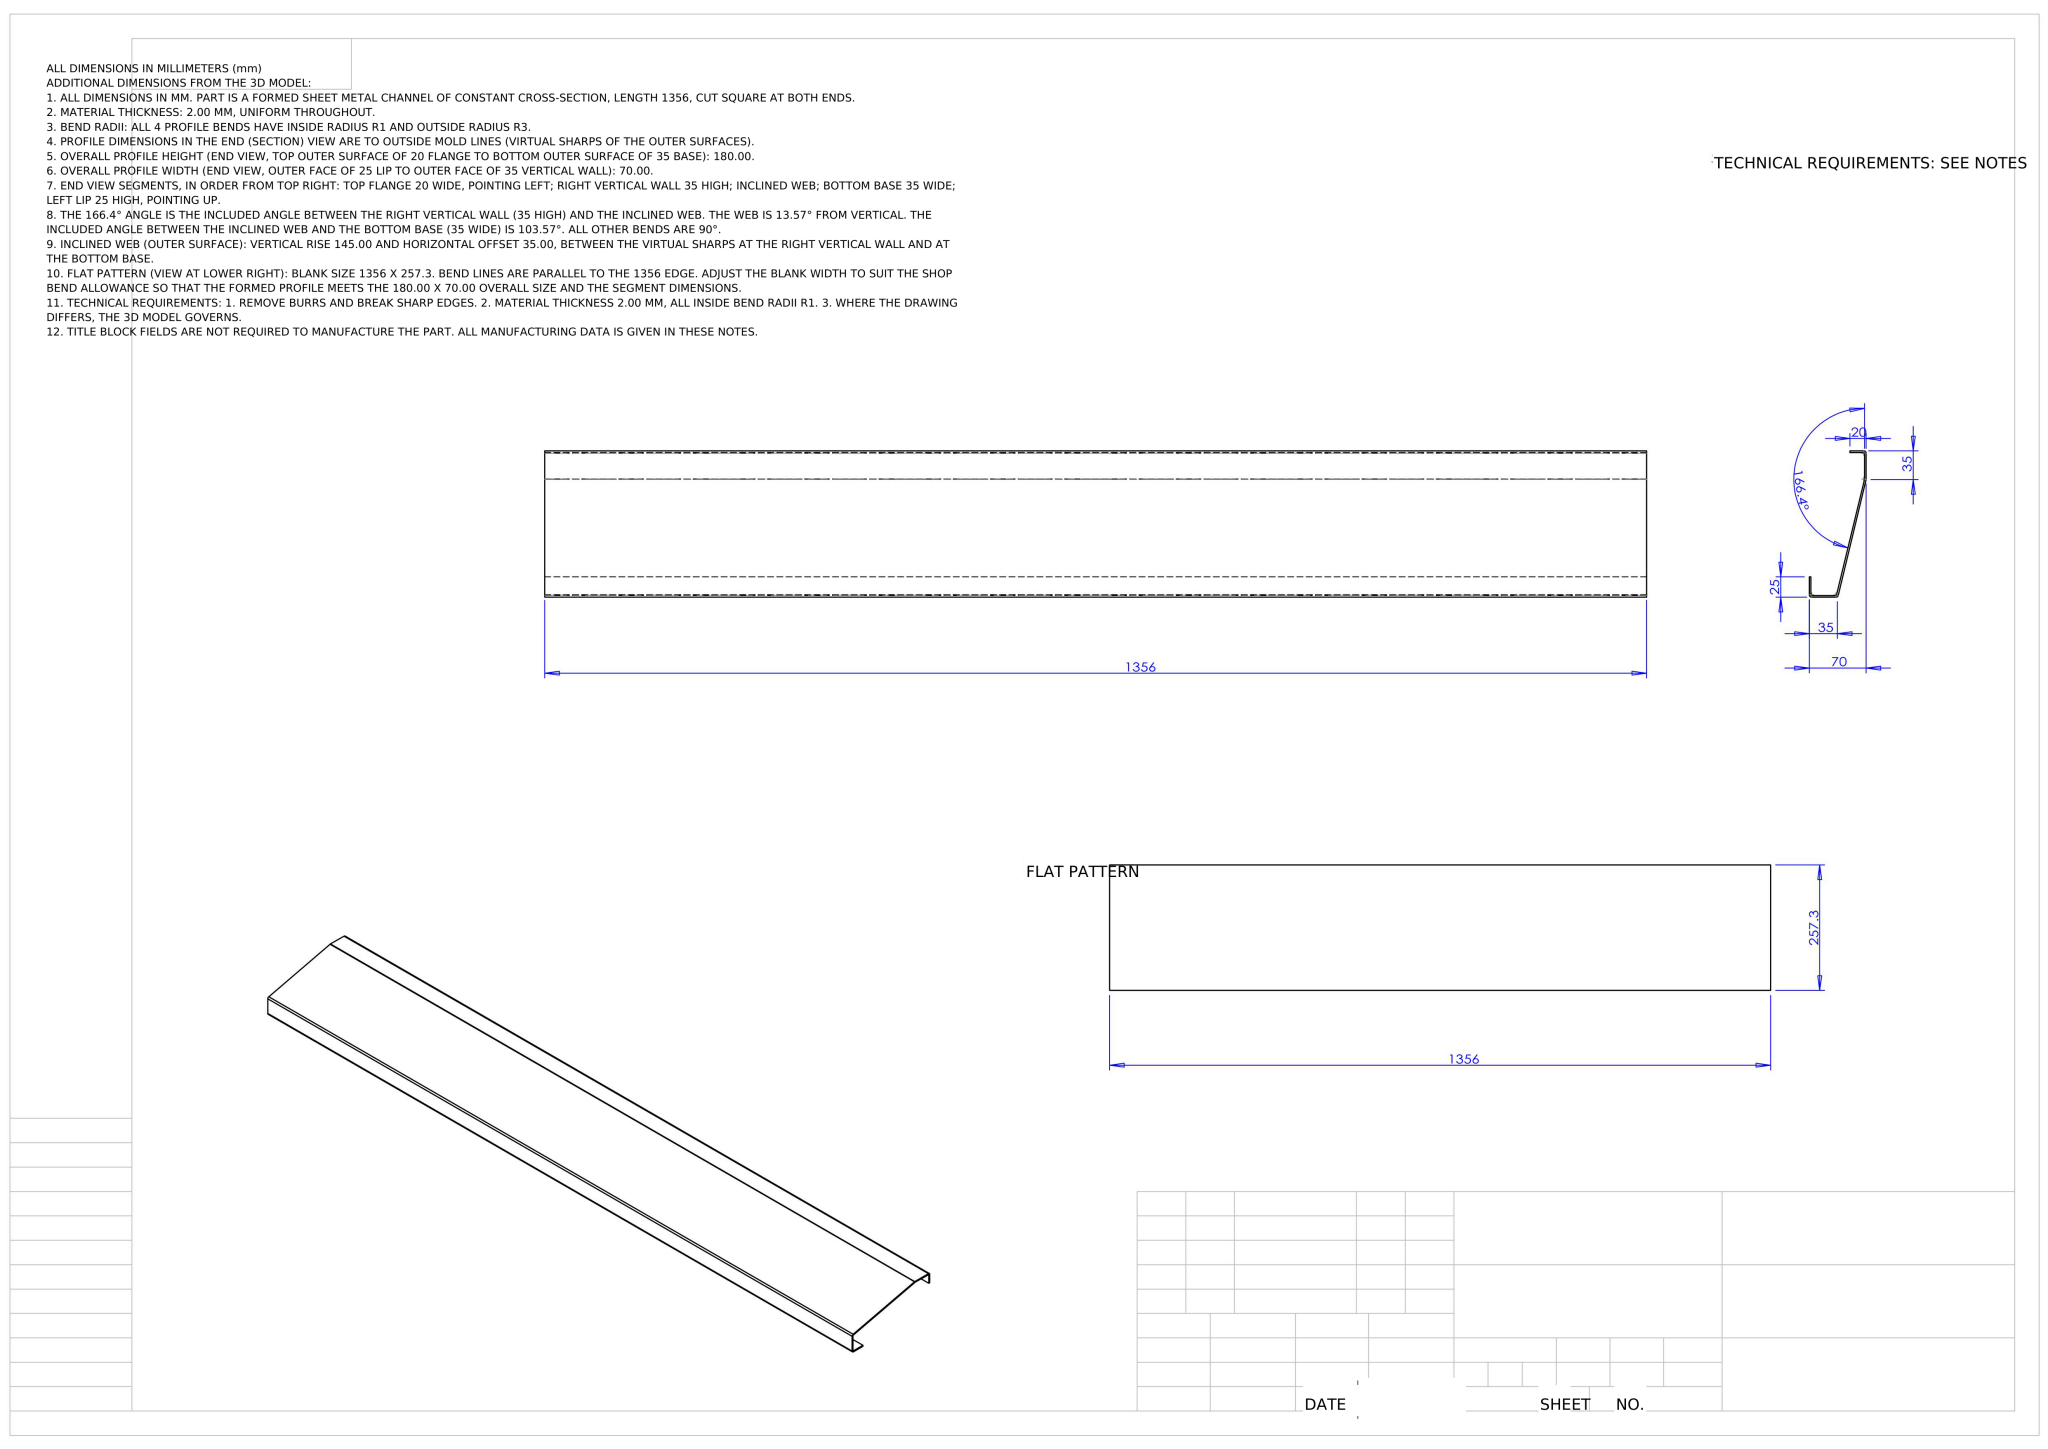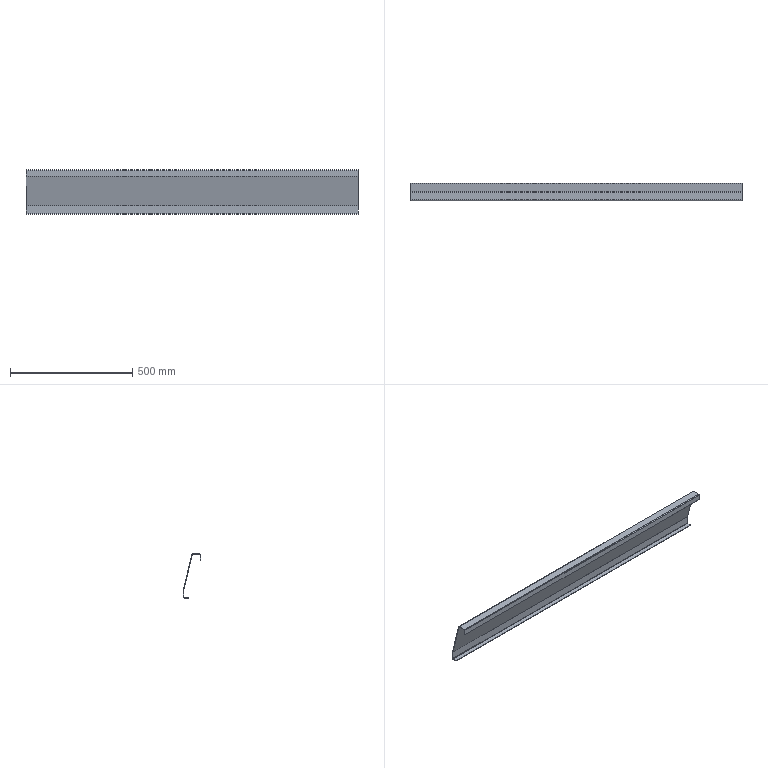Part | NX | mm | 1 solid | 38 faces | box 1356 x 70 x 180 mm | volume 694682 mm3 | plane 30 | cylinder 8 | commonest cylinder face diameters 2 x4 6 x4
STEP:
#1=COLOUR_RGB('',0.7529,0.7529,0.7529);
#2=FILL_AREA_STYLE_COLOUR('',#1);
#3=FILL_AREA_STYLE('',(#2));
#4=SURFACE_STYLE_FILL_AREA(#3);
#5=SURFACE_SIDE_STYLE('',(#4));
#6=SURFACE_STYLE_USAGE(.BOTH.,#5);
#7=PRESENTATION_STYLE_ASSIGNMENT((#6));
#8=CARTESIAN_POINT('',(1356.,-0.06513,-82.562));
#9=VERTEX_POINT('',#8);
#10=CARTESIAN_POINT('',(1356.,-0.06513,-80.562));
#11=VERTEX_POINT('',#10);
#12=CARTESIAN_POINT('',(1356.,-0.06513,-82.562));
#13=DIRECTION('',(0.,-0.,1.));
#14=VECTOR('',#13,1000.);
#15=LINE('',#12,#14);
#16=EDGE_CURVE('',#9,#11,#15,.T.);
#17=ORIENTED_EDGE('',*,*,#16,.F.);
#18=CARTESIAN_POINT('',(1356.,2.935,-79.562));
#19=VERTEX_POINT('',#18);
#20=CARTESIAN_POINT('',(1356.,-0.06513,-79.562));
#21=DIRECTION('',(1.,0.,0.));
#22=DIRECTION('',(0.,0.,1.));
#23=AXIS2_PLACEMENT_3D('',#20,#21,#22);
#24=CIRCLE('',#23,3.);
#25=EDGE_CURVE('',#9,#19,#24,.T.);
#26=ORIENTED_EDGE('',*,*,#25,.T.);
#27=CARTESIAN_POINT('',(1356.,0.9349,-79.562));
#28=VERTEX_POINT('',#27);
#29=CARTESIAN_POINT('',(1356.,0.9349,-79.562));
#30=DIRECTION('',(0.,1.,0.));
#31=VECTOR('',#30,1000.);
#32=LINE('',#29,#31);
#33=EDGE_CURVE('',#28,#19,#32,.T.);
#34=ORIENTED_EDGE('',*,*,#33,.F.);
#35=CARTESIAN_POINT('',(1356.,-0.06513,-79.562));
#36=DIRECTION('',(1.,0.,0.));
#37=DIRECTION('',(0.,0.,-1.));
#38=AXIS2_PLACEMENT_3D('',#35,#36,#37);
#39=CIRCLE('',#38,1.);
#40=EDGE_CURVE('',#11,#28,#39,.T.);
#41=ORIENTED_EDGE('',*,*,#40,.F.);
#42=EDGE_LOOP('',(#17,#26,#34,#41));
#43=FACE_OUTER_BOUND('',#42,.T.);
#44=CARTESIAN_POINT('',(1356.,-0.06513,-82.562));
#45=DIRECTION('',(1.,0.,0.));
#46=DIRECTION('',(0.,0.,-1.));
#47=AXIS2_PLACEMENT_3D('',#44,#45,#46);
#48=PLANE('',#47);
#49=ADVANCED_FACE('',(#43),#48,.T.);
#50=CARTESIAN_POINT('',(1356.,-17.065,-82.562));
#51=VERTEX_POINT('',#50);
#52=CARTESIAN_POINT('',(1356.,-17.065,-82.562));
#53=DIRECTION('',(0.,1.,0.));
#54=VECTOR('',#53,1000.);
#55=LINE('',#52,#54);
#56=EDGE_CURVE('',#51,#9,#55,.T.);
#57=ORIENTED_EDGE('',*,*,#56,.T.);
#58=ORIENTED_EDGE('',*,*,#16,.T.);
#59=CARTESIAN_POINT('',(1356.,-17.065,-80.562));
#60=VERTEX_POINT('',#59);
#61=CARTESIAN_POINT('',(1356.,-17.065,-80.562));
#62=DIRECTION('',(0.,1.,0.));
#63=VECTOR('',#62,1000.);
#64=LINE('',#61,#63);
#65=EDGE_CURVE('',#60,#11,#64,.T.);
#66=ORIENTED_EDGE('',*,*,#65,.F.);
#67=CARTESIAN_POINT('',(1356.,-17.065,-82.562));
#68=DIRECTION('',(0.,0.,1.));
#69=VECTOR('',#68,1000.);
#70=LINE('',#67,#69);
#71=EDGE_CURVE('',#51,#60,#70,.T.);
#72=ORIENTED_EDGE('',*,*,#71,.F.);
#73=EDGE_LOOP('',(#57,#58,#66,#72));
#74=FACE_OUTER_BOUND('',#73,.T.);
#75=CARTESIAN_POINT('',(1356.,0.9349,-79.562));
#76=DIRECTION('',(1.,0.,0.));
#77=DIRECTION('',(0.,0.,-1.));
#78=AXIS2_PLACEMENT_3D('',#75,#76,#77);
#79=PLANE('',#78);
#80=ADVANCED_FACE('',(#74),#79,.T.);
#81=CARTESIAN_POINT('',(0.,2.935,-79.562));
#82=VERTEX_POINT('',#81);
#83=CARTESIAN_POINT('',(0.,0.9349,-79.562));
#84=VERTEX_POINT('',#83);
#85=CARTESIAN_POINT('',(0.,2.935,-79.562));
#86=DIRECTION('',(0.,-1.,0.));
#87=VECTOR('',#86,1000.);
#88=LINE('',#85,#87);
#89=EDGE_CURVE('',#82,#84,#88,.T.);
#90=ORIENTED_EDGE('',*,*,#89,.F.);
#91=CARTESIAN_POINT('',(0.,-0.06513,-82.562));
#92=VERTEX_POINT('',#91);
#93=CARTESIAN_POINT('',(0.,-0.06513,-79.562));
#94=DIRECTION('',(1.,0.,0.));
#95=DIRECTION('',(0.,0.,1.));
#96=AXIS2_PLACEMENT_3D('',#93,#94,#95);
#97=CIRCLE('',#96,3.);
#98=EDGE_CURVE('',#92,#82,#97,.T.);
#99=ORIENTED_EDGE('',*,*,#98,.F.);
#100=CARTESIAN_POINT('',(0.,-0.06513,-80.562));
#101=VERTEX_POINT('',#100);
#102=CARTESIAN_POINT('',(0.,-0.06513,-80.562));
#103=DIRECTION('',(0.,0.,-1.));
#104=VECTOR('',#103,1000.);
#105=LINE('',#102,#104);
#106=EDGE_CURVE('',#101,#92,#105,.T.);
#107=ORIENTED_EDGE('',*,*,#106,.F.);
#108=CARTESIAN_POINT('',(0.,-0.06513,-79.562));
#109=DIRECTION('',(1.,0.,0.));
#110=DIRECTION('',(0.,0.,-1.));
#111=AXIS2_PLACEMENT_3D('',#108,#109,#110);
#112=CIRCLE('',#111,1.);
#113=EDGE_CURVE('',#101,#84,#112,.T.);
#114=ORIENTED_EDGE('',*,*,#113,.T.);
#115=EDGE_LOOP('',(#90,#99,#107,#114));
#116=FACE_OUTER_BOUND('',#115,.T.);
#117=CARTESIAN_POINT('',(0.,2.935,-79.562));
#118=DIRECTION('',(-1.,0.,0.));
#119=DIRECTION('',(0.,0.,1.));
#120=AXIS2_PLACEMENT_3D('',#117,#118,#119);
#121=PLANE('',#120);
#122=ADVANCED_FACE('',(#116),#121,.T.);
#123=CARTESIAN_POINT('',(0.,2.935,-47.919));
#124=VERTEX_POINT('',#123);
#125=CARTESIAN_POINT('',(0.,2.935,-82.562));
#126=DIRECTION('',(0.,-0.,1.));
#127=VECTOR('',#126,1000.);
#128=LINE('',#125,#127);
#129=EDGE_CURVE('',#82,#124,#128,.T.);
#130=ORIENTED_EDGE('',*,*,#129,.F.);
#131=ORIENTED_EDGE('',*,*,#89,.T.);
#132=CARTESIAN_POINT('',(0.,0.9349,-47.919));
#133=VERTEX_POINT('',#132);
#134=CARTESIAN_POINT('',(0.,0.9349,-82.562));
#135=DIRECTION('',(0.,-0.,1.));
#136=VECTOR('',#135,1000.);
#137=LINE('',#134,#136);
#138=EDGE_CURVE('',#84,#133,#137,.T.);
#139=ORIENTED_EDGE('',*,*,#138,.T.);
#140=CARTESIAN_POINT('',(0.,0.9349,-47.919));
#141=DIRECTION('',(0.,1.,0.));
#142=VECTOR('',#141,1000.);
#143=LINE('',#140,#142);
#144=EDGE_CURVE('',#133,#124,#143,.T.);
#145=ORIENTED_EDGE('',*,*,#144,.T.);
#146=EDGE_LOOP('',(#130,#131,#139,#145));
#147=FACE_OUTER_BOUND('',#146,.T.);
#148=CARTESIAN_POINT('',(0.,-0.06513,-80.562));
#149=DIRECTION('',(-1.,0.,0.));
#150=DIRECTION('',(0.,0.,1.));
#151=AXIS2_PLACEMENT_3D('',#148,#149,#150);
#152=PLANE('',#151);
#153=ADVANCED_FACE('',(#147),#152,.T.);
#154=CARTESIAN_POINT('',(1356.,2.935,-47.919));
#155=VERTEX_POINT('',#154);
#156=CARTESIAN_POINT('',(1356.,0.9349,-47.919));
#157=VERTEX_POINT('',#156);
#158=CARTESIAN_POINT('',(1356.,2.935,-47.919));
#159=DIRECTION('',(0.,-1.,0.));
#160=VECTOR('',#159,1000.);
#161=LINE('',#158,#160);
#162=EDGE_CURVE('',#155,#157,#161,.T.);
#163=ORIENTED_EDGE('',*,*,#162,.F.);
#164=CARTESIAN_POINT('',(1356.,2.851,-47.215));
#165=VERTEX_POINT('',#164);
#166=CARTESIAN_POINT('',(1356.,-0.06513,-47.919));
#167=DIRECTION('',(1.,0.,0.));
#168=DIRECTION('',(0.,-0.,1.));
#169=AXIS2_PLACEMENT_3D('',#166,#167,#168);
#170=CIRCLE('',#169,3.);
#171=EDGE_CURVE('',#155,#165,#170,.T.);
#172=ORIENTED_EDGE('',*,*,#171,.T.);
#173=CARTESIAN_POINT('',(1356.,0.907,-47.684));
#174=VERTEX_POINT('',#173);
#175=CARTESIAN_POINT('',(1356.,0.907,-47.684));
#176=DIRECTION('',(0.,0.9721,0.2346));
#177=VECTOR('',#176,1000.);
#178=LINE('',#175,#177);
#179=EDGE_CURVE('',#174,#165,#178,.T.);
#180=ORIENTED_EDGE('',*,*,#179,.F.);
#181=CARTESIAN_POINT('',(1356.,-0.06513,-47.919));
#182=DIRECTION('',(1.,0.,0.));
#183=DIRECTION('',(0.,0.,-1.));
#184=AXIS2_PLACEMENT_3D('',#181,#182,#183);
#185=CIRCLE('',#184,1.);
#186=EDGE_CURVE('',#157,#174,#185,.T.);
#187=ORIENTED_EDGE('',*,*,#186,.F.);
#188=EDGE_LOOP('',(#163,#172,#180,#187));
#189=FACE_OUTER_BOUND('',#188,.T.);
#190=CARTESIAN_POINT('',(1356.,2.935,-47.919));
#191=DIRECTION('',(1.,0.,0.));
#192=DIRECTION('',(0.,0.,-1.));
#193=AXIS2_PLACEMENT_3D('',#190,#191,#192);
#194=PLANE('',#193);
#195=ADVANCED_FACE('',(#189),#194,.T.);
#196=CARTESIAN_POINT('',(1356.,2.935,-82.562));
#197=DIRECTION('',(0.,-0.,1.));
#198=VECTOR('',#197,1000.);
#199=LINE('',#196,#198);
#200=EDGE_CURVE('',#19,#155,#199,.T.);
#201=ORIENTED_EDGE('',*,*,#200,.T.);
#202=ORIENTED_EDGE('',*,*,#162,.T.);
#203=CARTESIAN_POINT('',(1356.,0.9349,-82.562));
#204=DIRECTION('',(0.,-0.,1.));
#205=VECTOR('',#204,1000.);
#206=LINE('',#203,#205);
#207=EDGE_CURVE('',#28,#157,#206,.T.);
#208=ORIENTED_EDGE('',*,*,#207,.F.);
#209=ORIENTED_EDGE('',*,*,#33,.T.);
#210=EDGE_LOOP('',(#201,#202,#208,#209));
#211=FACE_OUTER_BOUND('',#210,.T.);
#212=CARTESIAN_POINT('',(1356.,0.907,-47.684));
#213=DIRECTION('',(1.,0.,0.));
#214=DIRECTION('',(0.,0.,-1.));
#215=AXIS2_PLACEMENT_3D('',#212,#213,#214);
#216=PLANE('',#215);
#217=ADVANCED_FACE('',(#211),#216,.T.);
#218=CARTESIAN_POINT('',(0.,2.851,-47.215));
#219=VERTEX_POINT('',#218);
#220=CARTESIAN_POINT('',(0.,0.907,-47.684));
#221=VERTEX_POINT('',#220);
#222=CARTESIAN_POINT('',(0.,2.851,-47.215));
#223=DIRECTION('',(0.,-0.9721,-0.2346));
#224=VECTOR('',#223,1000.);
#225=LINE('',#222,#224);
#226=EDGE_CURVE('',#219,#221,#225,.T.);
#227=ORIENTED_EDGE('',*,*,#226,.F.);
#228=CARTESIAN_POINT('',(0.,-0.06513,-47.919));
#229=DIRECTION('',(1.,0.,0.));
#230=DIRECTION('',(0.,-0.,1.));
#231=AXIS2_PLACEMENT_3D('',#228,#229,#230);
#232=CIRCLE('',#231,3.);
#233=EDGE_CURVE('',#124,#219,#232,.T.);
#234=ORIENTED_EDGE('',*,*,#233,.F.);
#235=ORIENTED_EDGE('',*,*,#144,.F.);
#236=CARTESIAN_POINT('',(0.,-0.06513,-47.919));
#237=DIRECTION('',(1.,0.,0.));
#238=DIRECTION('',(0.,0.,-1.));
#239=AXIS2_PLACEMENT_3D('',#236,#237,#238);
#240=CIRCLE('',#239,1.);
#241=EDGE_CURVE('',#133,#221,#240,.T.);
#242=ORIENTED_EDGE('',*,*,#241,.T.);
#243=EDGE_LOOP('',(#227,#234,#235,#242));
#244=FACE_OUTER_BOUND('',#243,.T.);
#245=CARTESIAN_POINT('',(0.,2.851,-47.215));
#246=DIRECTION('',(-1.,0.,0.));
#247=DIRECTION('',(0.,0.,1.));
#248=AXIS2_PLACEMENT_3D('',#245,#246,#247);
#249=PLANE('',#248);
#250=ADVANCED_FACE('',(#244),#249,.T.);
#251=CARTESIAN_POINT('',(0.,-31.511,95.142));
#252=VERTEX_POINT('',#251);
#253=CARTESIAN_POINT('',(0.,2.935,-47.562));
#254=DIRECTION('',(0.,-0.2346,0.9721));
#255=VECTOR('',#254,1000.);
#256=LINE('',#253,#255);
#257=EDGE_CURVE('',#219,#252,#256,.T.);
#258=ORIENTED_EDGE('',*,*,#257,.F.);
#259=ORIENTED_EDGE('',*,*,#226,.T.);
#260=CARTESIAN_POINT('',(0.,-33.455,94.672));
#261=VERTEX_POINT('',#260);
#262=CARTESIAN_POINT('',(0.,0.9907,-48.031));
#263=DIRECTION('',(0.,-0.2346,0.9721));
#264=VECTOR('',#263,1000.);
#265=LINE('',#262,#264);
#266=EDGE_CURVE('',#221,#261,#265,.T.);
#267=ORIENTED_EDGE('',*,*,#266,.T.);
#268=CARTESIAN_POINT('',(0.,-33.455,94.672));
#269=DIRECTION('',(0.,0.9721,0.2346));
#270=VECTOR('',#269,1000.);
#271=LINE('',#268,#270);
#272=EDGE_CURVE('',#261,#252,#271,.T.);
#273=ORIENTED_EDGE('',*,*,#272,.T.);
#274=EDGE_LOOP('',(#258,#259,#267,#273));
#275=FACE_OUTER_BOUND('',#274,.T.);
#276=CARTESIAN_POINT('',(0.,0.9349,-47.919));
#277=DIRECTION('',(-1.,0.,0.));
#278=DIRECTION('',(0.,0.,1.));
#279=AXIS2_PLACEMENT_3D('',#276,#277,#278);
#280=PLANE('',#279);
#281=ADVANCED_FACE('',(#275),#280,.T.);
#282=CARTESIAN_POINT('',(1356.,-31.511,95.142));
#283=VERTEX_POINT('',#282);
#284=CARTESIAN_POINT('',(1356.,-33.455,94.672));
#285=VERTEX_POINT('',#284);
#286=CARTESIAN_POINT('',(1356.,-31.511,95.142));
#287=DIRECTION('',(0.,-0.9721,-0.2346));
#288=VECTOR('',#287,1000.);
#289=LINE('',#286,#288);
#290=EDGE_CURVE('',#283,#285,#289,.T.);
#291=ORIENTED_EDGE('',*,*,#290,.F.);
#292=CARTESIAN_POINT('',(1356.,-34.427,97.438));
#293=VERTEX_POINT('',#292);
#294=CARTESIAN_POINT('',(1356.,-34.427,94.438));
#295=DIRECTION('',(1.,0.,0.));
#296=DIRECTION('',(0.,0.,1.));
#297=AXIS2_PLACEMENT_3D('',#294,#295,#296);
#298=CIRCLE('',#297,3.);
#299=EDGE_CURVE('',#283,#293,#298,.T.);
#300=ORIENTED_EDGE('',*,*,#299,.T.);
#301=CARTESIAN_POINT('',(1356.,-34.427,95.438));
#302=VERTEX_POINT('',#301);
#303=CARTESIAN_POINT('',(1356.,-34.427,95.438));
#304=DIRECTION('',(0.,0.,1.));
#305=VECTOR('',#304,1000.);
#306=LINE('',#303,#305);
#307=EDGE_CURVE('',#302,#293,#306,.T.);
#308=ORIENTED_EDGE('',*,*,#307,.F.);
#309=CARTESIAN_POINT('',(1356.,-34.427,94.438));
#310=DIRECTION('',(1.,0.,0.));
#311=DIRECTION('',(0.,0.,-1.));
#312=AXIS2_PLACEMENT_3D('',#309,#310,#311);
#313=CIRCLE('',#312,1.);
#314=EDGE_CURVE('',#285,#302,#313,.T.);
#315=ORIENTED_EDGE('',*,*,#314,.F.);
#316=EDGE_LOOP('',(#291,#300,#308,#315));
#317=FACE_OUTER_BOUND('',#316,.T.);
#318=CARTESIAN_POINT('',(1356.,-31.511,95.142));
#319=DIRECTION('',(1.,0.,0.));
#320=DIRECTION('',(0.,0.,-1.));
#321=AXIS2_PLACEMENT_3D('',#318,#319,#320);
#322=PLANE('',#321);
#323=ADVANCED_FACE('',(#317),#322,.T.);
#324=CARTESIAN_POINT('',(1356.,2.935,-47.562));
#325=DIRECTION('',(0.,-0.2346,0.9721));
#326=VECTOR('',#325,1000.);
#327=LINE('',#324,#326);
#328=EDGE_CURVE('',#165,#283,#327,.T.);
#329=ORIENTED_EDGE('',*,*,#328,.T.);
#330=ORIENTED_EDGE('',*,*,#290,.T.);
#331=CARTESIAN_POINT('',(1356.,0.9907,-48.031));
#332=DIRECTION('',(0.,-0.2346,0.9721));
#333=VECTOR('',#332,1000.);
#334=LINE('',#331,#333);
#335=EDGE_CURVE('',#174,#285,#334,.T.);
#336=ORIENTED_EDGE('',*,*,#335,.F.);
#337=ORIENTED_EDGE('',*,*,#179,.T.);
#338=EDGE_LOOP('',(#329,#330,#336,#337));
#339=FACE_OUTER_BOUND('',#338,.T.);
#340=CARTESIAN_POINT('',(1356.,-34.427,95.438));
#341=DIRECTION('',(1.,0.,0.));
#342=DIRECTION('',(0.,0.,-1.));
#343=AXIS2_PLACEMENT_3D('',#340,#341,#342);
#344=PLANE('',#343);
#345=ADVANCED_FACE('',(#339),#344,.T.);
#346=CARTESIAN_POINT('',(0.,-34.427,97.438));
#347=VERTEX_POINT('',#346);
#348=CARTESIAN_POINT('',(0.,-34.427,95.438));
#349=VERTEX_POINT('',#348);
#350=CARTESIAN_POINT('',(0.,-34.427,97.438));
#351=DIRECTION('',(0.,0.,-1.));
#352=VECTOR('',#351,1000.);
#353=LINE('',#350,#352);
#354=EDGE_CURVE('',#347,#349,#353,.T.);
#355=ORIENTED_EDGE('',*,*,#354,.F.);
#356=CARTESIAN_POINT('',(0.,-34.427,94.438));
#357=DIRECTION('',(1.,0.,0.));
#358=DIRECTION('',(0.,0.,1.));
#359=AXIS2_PLACEMENT_3D('',#356,#357,#358);
#360=CIRCLE('',#359,3.);
#361=EDGE_CURVE('',#252,#347,#360,.T.);
#362=ORIENTED_EDGE('',*,*,#361,.F.);
#363=ORIENTED_EDGE('',*,*,#272,.F.);
#364=CARTESIAN_POINT('',(0.,-34.427,94.438));
#365=DIRECTION('',(1.,0.,0.));
#366=DIRECTION('',(0.,0.,-1.));
#367=AXIS2_PLACEMENT_3D('',#364,#365,#366);
#368=CIRCLE('',#367,1.);
#369=EDGE_CURVE('',#261,#349,#368,.T.);
#370=ORIENTED_EDGE('',*,*,#369,.T.);
#371=EDGE_LOOP('',(#355,#362,#363,#370));
#372=FACE_OUTER_BOUND('',#371,.T.);
#373=CARTESIAN_POINT('',(0.,-34.427,97.438));
#374=DIRECTION('',(-1.,0.,0.));
#375=DIRECTION('',(0.,0.,1.));
#376=AXIS2_PLACEMENT_3D('',#373,#374,#375);
#377=PLANE('',#376);
#378=ADVANCED_FACE('',(#372),#377,.T.);
#379=CARTESIAN_POINT('',(0.,-64.065,97.438));
#380=VERTEX_POINT('',#379);
#381=CARTESIAN_POINT('',(0.,-32.065,97.438));
#382=DIRECTION('',(0.,-1.,0.));
#383=VECTOR('',#382,1000.);
#384=LINE('',#381,#383);
#385=EDGE_CURVE('',#347,#380,#384,.T.);
#386=ORIENTED_EDGE('',*,*,#385,.F.);
#387=ORIENTED_EDGE('',*,*,#354,.T.);
#388=CARTESIAN_POINT('',(0.,-64.065,95.438));
#389=VERTEX_POINT('',#388);
#390=CARTESIAN_POINT('',(0.,-32.065,95.438));
#391=DIRECTION('',(0.,-1.,0.));
#392=VECTOR('',#391,1000.);
#393=LINE('',#390,#392);
#394=EDGE_CURVE('',#349,#389,#393,.T.);
#395=ORIENTED_EDGE('',*,*,#394,.T.);
#396=CARTESIAN_POINT('',(0.,-64.065,95.438));
#397=DIRECTION('',(0.,0.,1.));
#398=VECTOR('',#397,1000.);
#399=LINE('',#396,#398);
#400=EDGE_CURVE('',#389,#380,#399,.T.);
#401=ORIENTED_EDGE('',*,*,#400,.T.);
#402=EDGE_LOOP('',(#386,#387,#395,#401));
#403=FACE_OUTER_BOUND('',#402,.T.);
#404=CARTESIAN_POINT('',(0.,-33.455,94.672));
#405=DIRECTION('',(-1.,0.,0.));
#406=DIRECTION('',(0.,0.,1.));
#407=AXIS2_PLACEMENT_3D('',#404,#405,#406);
#408=PLANE('',#407);
#409=ADVANCED_FACE('',(#403),#408,.T.);
#410=CARTESIAN_POINT('',(1356.,-64.065,97.438));
#411=VERTEX_POINT('',#410);
#412=CARTESIAN_POINT('',(1356.,-64.065,95.438));
#413=VERTEX_POINT('',#412);
#414=CARTESIAN_POINT('',(1356.,-64.065,97.438));
#415=DIRECTION('',(0.,0.,-1.));
#416=VECTOR('',#415,1000.);
#417=LINE('',#414,#416);
#418=EDGE_CURVE('',#411,#413,#417,.T.);
#419=ORIENTED_EDGE('',*,*,#418,.F.);
#420=CARTESIAN_POINT('',(1356.,-67.065,94.438));
#421=VERTEX_POINT('',#420);
#422=CARTESIAN_POINT('',(1356.,-64.065,94.438));
#423=DIRECTION('',(1.,0.,0.));
#424=DIRECTION('',(0.,0.,1.));
#425=AXIS2_PLACEMENT_3D('',#422,#423,#424);
#426=CIRCLE('',#425,3.);
#427=EDGE_CURVE('',#411,#421,#426,.T.);
#428=ORIENTED_EDGE('',*,*,#427,.T.);
#429=CARTESIAN_POINT('',(1356.,-65.065,94.438));
#430=VERTEX_POINT('',#429);
#431=CARTESIAN_POINT('',(1356.,-65.065,94.438));
#432=DIRECTION('',(0.,-1.,0.));
#433=VECTOR('',#432,1000.);
#434=LINE('',#431,#433);
#435=EDGE_CURVE('',#430,#421,#434,.T.);
#436=ORIENTED_EDGE('',*,*,#435,.F.);
#437=CARTESIAN_POINT('',(1356.,-64.065,94.438));
#438=DIRECTION('',(1.,0.,0.));
#439=DIRECTION('',(0.,0.,-1.));
#440=AXIS2_PLACEMENT_3D('',#437,#438,#439);
#441=CIRCLE('',#440,1.);
#442=EDGE_CURVE('',#413,#430,#441,.T.);
#443=ORIENTED_EDGE('',*,*,#442,.F.);
#444=EDGE_LOOP('',(#419,#428,#436,#443));
#445=FACE_OUTER_BOUND('',#444,.T.);
#446=CARTESIAN_POINT('',(1356.,-64.065,97.438));
#447=DIRECTION('',(1.,0.,0.));
#448=DIRECTION('',(0.,0.,-1.));
#449=AXIS2_PLACEMENT_3D('',#446,#447,#448);
#450=PLANE('',#449);
#451=ADVANCED_FACE('',(#445),#450,.T.);
#452=CARTESIAN_POINT('',(1356.,-32.065,97.438));
#453=DIRECTION('',(0.,-1.,0.));
#454=VECTOR('',#453,1000.);
#455=LINE('',#452,#454);
#456=EDGE_CURVE('',#293,#411,#455,.T.);
#457=ORIENTED_EDGE('',*,*,#456,.T.);
#458=ORIENTED_EDGE('',*,*,#418,.T.);
#459=CARTESIAN_POINT('',(1356.,-32.065,95.438));
#460=DIRECTION('',(0.,-1.,0.));
#461=VECTOR('',#460,1000.);
#462=LINE('',#459,#461);
#463=EDGE_CURVE('',#302,#413,#462,.T.);
#464=ORIENTED_EDGE('',*,*,#463,.F.);
#465=ORIENTED_EDGE('',*,*,#307,.T.);
#466=EDGE_LOOP('',(#457,#458,#464,#465));
#467=FACE_OUTER_BOUND('',#466,.T.);
#468=CARTESIAN_POINT('',(1356.,-65.065,94.438));
#469=DIRECTION('',(1.,0.,0.));
#470=DIRECTION('',(0.,0.,-1.));
#471=AXIS2_PLACEMENT_3D('',#468,#469,#470);
#472=PLANE('',#471);
#473=ADVANCED_FACE('',(#467),#472,.T.);
#474=CARTESIAN_POINT('',(0.,-67.065,94.438));
#475=VERTEX_POINT('',#474);
#476=CARTESIAN_POINT('',(0.,-65.065,94.438));
#477=VERTEX_POINT('',#476);
#478=CARTESIAN_POINT('',(0.,-67.065,94.438));
#479=DIRECTION('',(0.,1.,0.));
#480=VECTOR('',#479,1000.);
#481=LINE('',#478,#480);
#482=EDGE_CURVE('',#475,#477,#481,.T.);
#483=ORIENTED_EDGE('',*,*,#482,.F.);
#484=CARTESIAN_POINT('',(0.,-64.065,94.438));
#485=DIRECTION('',(1.,0.,0.));
#486=DIRECTION('',(0.,0.,1.));
#487=AXIS2_PLACEMENT_3D('',#484,#485,#486);
#488=CIRCLE('',#487,3.);
#489=EDGE_CURVE('',#380,#475,#488,.T.);
#490=ORIENTED_EDGE('',*,*,#489,.F.);
#491=ORIENTED_EDGE('',*,*,#400,.F.);
#492=CARTESIAN_POINT('',(0.,-64.065,94.438));
#493=DIRECTION('',(1.,0.,0.));
#494=DIRECTION('',(0.,0.,-1.));
#495=AXIS2_PLACEMENT_3D('',#492,#493,#494);
#496=CIRCLE('',#495,1.);
#497=EDGE_CURVE('',#389,#477,#496,.T.);
#498=ORIENTED_EDGE('',*,*,#497,.T.);
#499=EDGE_LOOP('',(#483,#490,#491,#498));
#500=FACE_OUTER_BOUND('',#499,.T.);
#501=CARTESIAN_POINT('',(0.,-67.065,94.438));
#502=DIRECTION('',(-1.,0.,0.));
#503=DIRECTION('',(0.,0.,1.));
#504=AXIS2_PLACEMENT_3D('',#501,#502,#503);
#505=PLANE('',#504);
#506=ADVANCED_FACE('',(#500),#505,.T.);
#507=CARTESIAN_POINT('',(0.,-67.065,72.438));
#508=VERTEX_POINT('',#507);
#509=CARTESIAN_POINT('',(0.,-67.065,97.438));
#510=DIRECTION('',(0.,0.,-1.));
#511=VECTOR('',#510,1000.);
#512=LINE('',#509,#511);
#513=EDGE_CURVE('',#475,#508,#512,.T.);
#514=ORIENTED_EDGE('',*,*,#513,.F.);
#515=ORIENTED_EDGE('',*,*,#482,.T.);
#516=CARTESIAN_POINT('',(0.,-65.065,72.438));
#517=VERTEX_POINT('',#516);
#518=CARTESIAN_POINT('',(0.,-65.065,97.438));
#519=DIRECTION('',(0.,0.,-1.));
#520=VECTOR('',#519,1000.);
#521=LINE('',#518,#520);
#522=EDGE_CURVE('',#477,#517,#521,.T.);
#523=ORIENTED_EDGE('',*,*,#522,.T.);
#524=CARTESIAN_POINT('',(0.,-65.065,72.438));
#525=DIRECTION('',(0.,-1.,0.));
#526=VECTOR('',#525,1000.);
#527=LINE('',#524,#526);
#528=EDGE_CURVE('',#517,#508,#527,.T.);
#529=ORIENTED_EDGE('',*,*,#528,.T.);
#530=EDGE_LOOP('',(#514,#515,#523,#529));
#531=FACE_OUTER_BOUND('',#530,.T.);
#532=CARTESIAN_POINT('',(0.,-64.065,95.438));
#533=DIRECTION('',(-1.,0.,0.));
#534=DIRECTION('',(0.,0.,1.));
#535=AXIS2_PLACEMENT_3D('',#532,#533,#534);
#536=PLANE('',#535);
#537=ADVANCED_FACE('',(#531),#536,.T.);
#538=ORIENTED_EDGE('',*,*,#513,.T.);
#539=CARTESIAN_POINT('',(1356.,-67.065,72.438));
#540=VERTEX_POINT('',#539);
#541=CARTESIAN_POINT('',(1356.,-67.065,72.438));
#542=DIRECTION('',(-1.,0.,0.));
#543=VECTOR('',#542,1000.);
#544=LINE('',#541,#543);
#545=EDGE_CURVE('',#540,#508,#544,.T.);
#546=ORIENTED_EDGE('',*,*,#545,.F.);
#547=CARTESIAN_POINT('',(1356.,-67.065,97.438));
#548=DIRECTION('',(0.,0.,-1.));
#549=VECTOR('',#548,1000.);
#550=LINE('',#547,#549);
#551=EDGE_CURVE('',#421,#540,#550,.T.);
#552=ORIENTED_EDGE('',*,*,#551,.F.);
#553=CARTESIAN_POINT('',(1356.,-67.065,94.438));
#554=DIRECTION('',(-1.,0.,0.));
#555=VECTOR('',#554,1000.);
#556=LINE('',#553,#555);
#557=EDGE_CURVE('',#421,#475,#556,.T.);
#558=ORIENTED_EDGE('',*,*,#557,.T.);
#559=EDGE_LOOP('',(#538,#546,#552,#558));
#560=FACE_OUTER_BOUND('',#559,.T.);
#561=CARTESIAN_POINT('',(1356.,-67.065,97.438));
#562=DIRECTION('',(0.,1.,0.));
#563=DIRECTION('',(0.,0.,1.));
#564=AXIS2_PLACEMENT_3D('',#561,#562,#563);
#565=PLANE('',#564);
#566=ADVANCED_FACE('',(#560),#565,.F.);
#567=ORIENTED_EDGE('',*,*,#528,.F.);
#568=CARTESIAN_POINT('',(1356.,-65.065,72.438));
#569=VERTEX_POINT('',#568);
#570=CARTESIAN_POINT('',(1356.,-65.065,72.438));
#571=DIRECTION('',(-1.,0.,0.));
#572=VECTOR('',#571,1000.);
#573=LINE('',#570,#572);
#574=EDGE_CURVE('',#569,#517,#573,.T.);
#575=ORIENTED_EDGE('',*,*,#574,.F.);
#576=CARTESIAN_POINT('',(1356.,-65.065,72.438));
#577=DIRECTION('',(0.,-1.,0.));
#578=VECTOR('',#577,1000.);
#579=LINE('',#576,#578);
#580=EDGE_CURVE('',#569,#540,#579,.T.);
#581=ORIENTED_EDGE('',*,*,#580,.T.);
#582=ORIENTED_EDGE('',*,*,#545,.T.);
#583=EDGE_LOOP('',(#567,#575,#581,#582));
#584=FACE_OUTER_BOUND('',#583,.T.);
#585=CARTESIAN_POINT('',(1356.,-65.065,72.438));
#586=DIRECTION('',(0.,0.,-1.));
#587=DIRECTION('',(-1.,0.,0.));
#588=AXIS2_PLACEMENT_3D('',#585,#586,#587);
#589=PLANE('',#588);
#590=ADVANCED_FACE('',(#584),#589,.T.);
#591=ORIENTED_EDGE('',*,*,#522,.F.);
#592=CARTESIAN_POINT('',(1356.,-65.065,94.438));
#593=DIRECTION('',(-1.,0.,0.));
#594=VECTOR('',#593,1000.);
#595=LINE('',#592,#594);
#596=EDGE_CURVE('',#430,#477,#595,.T.);
#597=ORIENTED_EDGE('',*,*,#596,.F.);
#598=CARTESIAN_POINT('',(1356.,-65.065,97.438));
#599=DIRECTION('',(0.,0.,-1.));
#600=VECTOR('',#599,1000.);
#601=LINE('',#598,#600);
#602=EDGE_CURVE('',#430,#569,#601,.T.);
#603=ORIENTED_EDGE('',*,*,#602,.T.);
#604=ORIENTED_EDGE('',*,*,#574,.T.);
#605=EDGE_LOOP('',(#591,#597,#603,#604));
#606=FACE_OUTER_BOUND('',#605,.T.);
#607=CARTESIAN_POINT('',(1356.,-65.065,97.438));
#608=DIRECTION('',(0.,1.,0.));
#609=DIRECTION('',(0.,0.,1.));
#610=AXIS2_PLACEMENT_3D('',#607,#608,#609);
#611=PLANE('',#610);
#612=ADVANCED_FACE('',(#606),#611,.T.);
#613=ORIENTED_EDGE('',*,*,#497,.F.);
#614=CARTESIAN_POINT('',(1356.,-64.065,95.438));
#615=DIRECTION('',(-1.,0.,0.));
#616=VECTOR('',#615,1000.);
#617=LINE('',#614,#616);
#618=EDGE_CURVE('',#413,#389,#617,.T.);
#619=ORIENTED_EDGE('',*,*,#618,.F.);
#620=ORIENTED_EDGE('',*,*,#442,.T.);
#621=ORIENTED_EDGE('',*,*,#596,.T.);
#622=EDGE_LOOP('',(#613,#619,#620,#621));
#623=FACE_OUTER_BOUND('',#622,.T.);
#624=CARTESIAN_POINT('',(1356.,-64.065,94.438));
#625=DIRECTION('',(-1.,0.,0.));
#626=DIRECTION('',(0.,0.,1.));
#627=AXIS2_PLACEMENT_3D('',#624,#625,#626);
#628=CYLINDRICAL_SURFACE('',#627,1.);
#629=ADVANCED_FACE('',(#623),#628,.F.);
#630=ORIENTED_EDGE('',*,*,#394,.F.);
#631=CARTESIAN_POINT('',(1356.,-34.427,95.438));
#632=DIRECTION('',(-1.,0.,0.));
#633=VECTOR('',#632,1000.);
#634=LINE('',#631,#633);
#635=EDGE_CURVE('',#302,#349,#634,.T.);
#636=ORIENTED_EDGE('',*,*,#635,.F.);
#637=ORIENTED_EDGE('',*,*,#463,.T.);
#638=ORIENTED_EDGE('',*,*,#618,.T.);
#639=EDGE_LOOP('',(#630,#636,#637,#638));
#640=FACE_OUTER_BOUND('',#639,.T.);
#641=CARTESIAN_POINT('',(1356.,-32.065,95.438));
#642=DIRECTION('',(0.,0.,-1.));
#643=DIRECTION('',(-1.,0.,0.));
#644=AXIS2_PLACEMENT_3D('',#641,#642,#643);
#645=PLANE('',#644);
#646=ADVANCED_FACE('',(#640),#645,.T.);
#647=ORIENTED_EDGE('',*,*,#369,.F.);
#648=CARTESIAN_POINT('',(1356.,-33.455,94.672));
#649=DIRECTION('',(-1.,0.,0.));
#650=VECTOR('',#649,1000.);
#651=LINE('',#648,#650);
#652=EDGE_CURVE('',#285,#261,#651,.T.);
#653=ORIENTED_EDGE('',*,*,#652,.F.);
#654=ORIENTED_EDGE('',*,*,#314,.T.);
#655=ORIENTED_EDGE('',*,*,#635,.T.);
#656=EDGE_LOOP('',(#647,#653,#654,#655));
#657=FACE_OUTER_BOUND('',#656,.T.);
#658=CARTESIAN_POINT('',(1356.,-34.427,94.438));
#659=DIRECTION('',(-1.,0.,0.));
#660=DIRECTION('',(0.,0.,1.));
#661=AXIS2_PLACEMENT_3D('',#658,#659,#660);
#662=CYLINDRICAL_SURFACE('',#661,1.);
#663=ADVANCED_FACE('',(#657),#662,.F.);
#664=ORIENTED_EDGE('',*,*,#266,.F.);
#665=CARTESIAN_POINT('',(1356.,0.907,-47.684));
#666=DIRECTION('',(-1.,0.,0.));
#667=VECTOR('',#666,1000.);
#668=LINE('',#665,#667);
#669=EDGE_CURVE('',#174,#221,#668,.T.);
#670=ORIENTED_EDGE('',*,*,#669,.F.);
#671=ORIENTED_EDGE('',*,*,#335,.T.);
#672=ORIENTED_EDGE('',*,*,#652,.T.);
#673=EDGE_LOOP('',(#664,#670,#671,#672));
#674=FACE_OUTER_BOUND('',#673,.T.);
#675=CARTESIAN_POINT('',(1356.,0.9907,-48.031));
#676=DIRECTION('',(0.,-0.9721,-0.2346));
#677=DIRECTION('',(0.,0.2346,-0.9721));
#678=AXIS2_PLACEMENT_3D('',#675,#676,#677);
#679=PLANE('',#678);
#680=ADVANCED_FACE('',(#674),#679,.T.);
#681=ORIENTED_EDGE('',*,*,#241,.F.);
#682=CARTESIAN_POINT('',(1356.,0.9349,-47.919));
#683=DIRECTION('',(-1.,0.,0.));
#684=VECTOR('',#683,1000.);
#685=LINE('',#682,#684);
#686=EDGE_CURVE('',#157,#133,#685,.T.);
#687=ORIENTED_EDGE('',*,*,#686,.F.);
#688=ORIENTED_EDGE('',*,*,#186,.T.);
#689=ORIENTED_EDGE('',*,*,#669,.T.);
#690=EDGE_LOOP('',(#681,#687,#688,#689));
#691=FACE_OUTER_BOUND('',#690,.T.);
#692=CARTESIAN_POINT('',(1356.,-0.06513,-47.919));
#693=DIRECTION('',(-1.,0.,0.));
#694=DIRECTION('',(0.,0.,1.));
#695=AXIS2_PLACEMENT_3D('',#692,#693,#694);
#696=CYLINDRICAL_SURFACE('',#695,1.);
#697=ADVANCED_FACE('',(#691),#696,.F.);
#698=ORIENTED_EDGE('',*,*,#138,.F.);
#699=CARTESIAN_POINT('',(1356.,0.9349,-79.562));
#700=DIRECTION('',(-1.,0.,0.));
#701=VECTOR('',#700,1000.);
#702=LINE('',#699,#701);
#703=EDGE_CURVE('',#28,#84,#702,.T.);
#704=ORIENTED_EDGE('',*,*,#703,.F.);
#705=ORIENTED_EDGE('',*,*,#207,.T.);
#706=ORIENTED_EDGE('',*,*,#686,.T.);
#707=EDGE_LOOP('',(#698,#704,#705,#706));
#708=FACE_OUTER_BOUND('',#707,.T.);
#709=CARTESIAN_POINT('',(1356.,0.9349,-82.562));
#710=DIRECTION('',(0.,-1.,-0.));
#711=DIRECTION('',(0.,0.,-1.));
#712=AXIS2_PLACEMENT_3D('',#709,#710,#711);
#713=PLANE('',#712);
#714=ADVANCED_FACE('',(#708),#713,.T.);
#715=ORIENTED_EDGE('',*,*,#113,.F.);
#716=CARTESIAN_POINT('',(1356.,-0.06513,-80.562));
#717=DIRECTION('',(-1.,0.,0.));
#718=VECTOR('',#717,1000.);
#719=LINE('',#716,#718);
#720=EDGE_CURVE('',#11,#101,#719,.T.);
#721=ORIENTED_EDGE('',*,*,#720,.F.);
#722=ORIENTED_EDGE('',*,*,#40,.T.);
#723=ORIENTED_EDGE('',*,*,#703,.T.);
#724=EDGE_LOOP('',(#715,#721,#722,#723));
#725=FACE_OUTER_BOUND('',#724,.T.);
#726=CARTESIAN_POINT('',(1356.,-0.06513,-79.562));
#727=DIRECTION('',(-1.,0.,0.));
#728=DIRECTION('',(0.,0.,1.));
#729=AXIS2_PLACEMENT_3D('',#726,#727,#728);
#730=CYLINDRICAL_SURFACE('',#729,1.);
#731=ADVANCED_FACE('',(#725),#730,.F.);
#732=CARTESIAN_POINT('',(0.,-17.065,-80.562));
#733=VERTEX_POINT('',#732);
#734=CARTESIAN_POINT('',(0.,-17.065,-80.562));
#735=DIRECTION('',(0.,1.,0.));
#736=VECTOR('',#735,1000.);
#737=LINE('',#734,#736);
#738=EDGE_CURVE('',#733,#101,#737,.T.);
#739=ORIENTED_EDGE('',*,*,#738,.F.);
#740=CARTESIAN_POINT('',(1356.,-17.065,-80.562));
#741=DIRECTION('',(-1.,0.,0.));
#742=VECTOR('',#741,1000.);
#743=LINE('',#740,#742);
#744=EDGE_CURVE('',#60,#733,#743,.T.);
#745=ORIENTED_EDGE('',*,*,#744,.F.);
#746=ORIENTED_EDGE('',*,*,#65,.T.);
#747=ORIENTED_EDGE('',*,*,#720,.T.);
#748=EDGE_LOOP('',(#739,#745,#746,#747));
#749=FACE_OUTER_BOUND('',#748,.T.);
#750=CARTESIAN_POINT('',(1356.,-17.065,-80.562));
#751=DIRECTION('',(0.,0.,1.));
#752=DIRECTION('',(1.,0.,0.));
#753=AXIS2_PLACEMENT_3D('',#750,#751,#752);
#754=PLANE('',#753);
#755=ADVANCED_FACE('',(#749),#754,.T.);
#756=CARTESIAN_POINT('',(0.,-17.065,-82.562));
#757=VERTEX_POINT('',#756);
#758=CARTESIAN_POINT('',(0.,-17.065,-82.562));
#759=DIRECTION('',(0.,0.,1.));
#760=VECTOR('',#759,1000.);
#761=LINE('',#758,#760);
#762=EDGE_CURVE('',#757,#733,#761,.T.);
#763=ORIENTED_EDGE('',*,*,#762,.F.);
#764=CARTESIAN_POINT('',(1356.,-17.065,-82.562));
#765=DIRECTION('',(-1.,0.,0.));
#766=VECTOR('',#765,1000.);
#767=LINE('',#764,#766);
#768=EDGE_CURVE('',#51,#757,#767,.T.);
#769=ORIENTED_EDGE('',*,*,#768,.F.);
#770=ORIENTED_EDGE('',*,*,#71,.T.);
#771=ORIENTED_EDGE('',*,*,#744,.T.);
#772=EDGE_LOOP('',(#763,#769,#770,#771));
#773=FACE_OUTER_BOUND('',#772,.T.);
#774=CARTESIAN_POINT('',(1356.,-17.065,-82.562));
#775=DIRECTION('',(0.,-1.,0.));
#776=DIRECTION('',(0.,0.,-1.));
#777=AXIS2_PLACEMENT_3D('',#774,#775,#776);
#778=PLANE('',#777);
#779=ADVANCED_FACE('',(#773),#778,.T.);
#780=CARTESIAN_POINT('',(0.,-17.065,-82.562));
#781=DIRECTION('',(0.,1.,0.));
#782=VECTOR('',#781,1000.);
#783=LINE('',#780,#782);
#784=EDGE_CURVE('',#757,#92,#783,.T.);
#785=ORIENTED_EDGE('',*,*,#784,.T.);
#786=CARTESIAN_POINT('',(1356.,-0.06513,-82.562));
#787=DIRECTION('',(-1.,0.,0.));
#788=VECTOR('',#787,1000.);
#789=LINE('',#786,#788);
#790=EDGE_CURVE('',#9,#92,#789,.T.);
#791=ORIENTED_EDGE('',*,*,#790,.F.);
#792=ORIENTED_EDGE('',*,*,#56,.F.);
#793=ORIENTED_EDGE('',*,*,#768,.T.);
#794=EDGE_LOOP('',(#785,#791,#792,#793));
#795=FACE_OUTER_BOUND('',#794,.T.);
#796=CARTESIAN_POINT('',(1356.,-17.065,-82.562));
#797=DIRECTION('',(0.,0.,1.));
#798=DIRECTION('',(1.,0.,0.));
#799=AXIS2_PLACEMENT_3D('',#796,#797,#798);
#800=PLANE('',#799);
#801=ADVANCED_FACE('',(#795),#800,.F.);
#802=ORIENTED_EDGE('',*,*,#98,.T.);
#803=CARTESIAN_POINT('',(1356.,2.935,-79.562));
#804=DIRECTION('',(-1.,0.,0.));
#805=VECTOR('',#804,1000.);
#806=LINE('',#803,#805);
#807=EDGE_CURVE('',#19,#82,#806,.T.);
#808=ORIENTED_EDGE('',*,*,#807,.F.);
#809=ORIENTED_EDGE('',*,*,#25,.F.);
#810=ORIENTED_EDGE('',*,*,#790,.T.);
#811=EDGE_LOOP('',(#802,#808,#809,#810));
#812=FACE_OUTER_BOUND('',#811,.T.);
#813=CARTESIAN_POINT('',(1356.,-0.06513,-79.562));
#814=DIRECTION('',(-1.,0.,0.));
#815=DIRECTION('',(0.,0.,1.));
#816=AXIS2_PLACEMENT_3D('',#813,#814,#815);
#817=CYLINDRICAL_SURFACE('',#816,3.);
#818=ADVANCED_FACE('',(#812),#817,.T.);
#819=ORIENTED_EDGE('',*,*,#129,.T.);
#820=CARTESIAN_POINT('',(1356.,2.935,-47.919));
#821=DIRECTION('',(-1.,0.,0.));
#822=VECTOR('',#821,1000.);
#823=LINE('',#820,#822);
#824=EDGE_CURVE('',#155,#124,#823,.T.);
#825=ORIENTED_EDGE('',*,*,#824,.F.);
#826=ORIENTED_EDGE('',*,*,#200,.F.);
#827=ORIENTED_EDGE('',*,*,#807,.T.);
#828=EDGE_LOOP('',(#819,#825,#826,#827));
#829=FACE_OUTER_BOUND('',#828,.T.);
#830=CARTESIAN_POINT('',(1356.,2.935,-82.562));
#831=DIRECTION('',(0.,-1.,-0.));
#832=DIRECTION('',(0.,0.,-1.));
#833=AXIS2_PLACEMENT_3D('',#830,#831,#832);
#834=PLANE('',#833);
#835=ADVANCED_FACE('',(#829),#834,.F.);
#836=ORIENTED_EDGE('',*,*,#233,.T.);
#837=CARTESIAN_POINT('',(1356.,2.851,-47.215));
#838=DIRECTION('',(-1.,0.,0.));
#839=VECTOR('',#838,1000.);
#840=LINE('',#837,#839);
#841=EDGE_CURVE('',#165,#219,#840,.T.);
#842=ORIENTED_EDGE('',*,*,#841,.F.);
#843=ORIENTED_EDGE('',*,*,#171,.F.);
#844=ORIENTED_EDGE('',*,*,#824,.T.);
#845=EDGE_LOOP('',(#836,#842,#843,#844));
#846=FACE_OUTER_BOUND('',#845,.T.);
#847=CARTESIAN_POINT('',(1356.,-0.06513,-47.919));
#848=DIRECTION('',(-1.,0.,0.));
#849=DIRECTION('',(0.,0.,1.));
#850=AXIS2_PLACEMENT_3D('',#847,#848,#849);
#851=CYLINDRICAL_SURFACE('',#850,3.);
#852=ADVANCED_FACE('',(#846),#851,.T.);
#853=ORIENTED_EDGE('',*,*,#257,.T.);
#854=CARTESIAN_POINT('',(1356.,-31.511,95.142));
#855=DIRECTION('',(-1.,0.,0.));
#856=VECTOR('',#855,1000.);
#857=LINE('',#854,#856);
#858=EDGE_CURVE('',#283,#252,#857,.T.);
#859=ORIENTED_EDGE('',*,*,#858,.F.);
#860=ORIENTED_EDGE('',*,*,#328,.F.);
#861=ORIENTED_EDGE('',*,*,#841,.T.);
#862=EDGE_LOOP('',(#853,#859,#860,#861));
#863=FACE_OUTER_BOUND('',#862,.T.);
#864=CARTESIAN_POINT('',(1356.,2.935,-47.562));
#865=DIRECTION('',(0.,-0.9721,-0.2346));
#866=DIRECTION('',(0.,0.2346,-0.9721));
#867=AXIS2_PLACEMENT_3D('',#864,#865,#866);
#868=PLANE('',#867);
#869=ADVANCED_FACE('',(#863),#868,.F.);
#870=ORIENTED_EDGE('',*,*,#361,.T.);
#871=CARTESIAN_POINT('',(1356.,-34.427,97.438));
#872=DIRECTION('',(-1.,0.,0.));
#873=VECTOR('',#872,1000.);
#874=LINE('',#871,#873);
#875=EDGE_CURVE('',#293,#347,#874,.T.);
#876=ORIENTED_EDGE('',*,*,#875,.F.);
#877=ORIENTED_EDGE('',*,*,#299,.F.);
#878=ORIENTED_EDGE('',*,*,#858,.T.);
#879=EDGE_LOOP('',(#870,#876,#877,#878));
#880=FACE_OUTER_BOUND('',#879,.T.);
#881=CARTESIAN_POINT('',(1356.,-34.427,94.438));
#882=DIRECTION('',(-1.,0.,0.));
#883=DIRECTION('',(0.,0.,1.));
#884=AXIS2_PLACEMENT_3D('',#881,#882,#883);
#885=CYLINDRICAL_SURFACE('',#884,3.);
#886=ADVANCED_FACE('',(#880),#885,.T.);
#887=ORIENTED_EDGE('',*,*,#385,.T.);
#888=CARTESIAN_POINT('',(1356.,-64.065,97.438));
#889=DIRECTION('',(-1.,0.,0.));
#890=VECTOR('',#889,1000.);
#891=LINE('',#888,#890);
#892=EDGE_CURVE('',#411,#380,#891,.T.);
#893=ORIENTED_EDGE('',*,*,#892,.F.);
#894=ORIENTED_EDGE('',*,*,#456,.F.);
#895=ORIENTED_EDGE('',*,*,#875,.T.);
#896=EDGE_LOOP('',(#887,#893,#894,#895));
#897=FACE_OUTER_BOUND('',#896,.T.);
#898=CARTESIAN_POINT('',(1356.,-32.065,97.438));
#899=DIRECTION('',(0.,0.,-1.));
#900=DIRECTION('',(-1.,0.,0.));
#901=AXIS2_PLACEMENT_3D('',#898,#899,#900);
#902=PLANE('',#901);
#903=ADVANCED_FACE('',(#897),#902,.F.);
#904=ORIENTED_EDGE('',*,*,#489,.T.);
#905=ORIENTED_EDGE('',*,*,#557,.F.);
#906=ORIENTED_EDGE('',*,*,#427,.F.);
#907=ORIENTED_EDGE('',*,*,#892,.T.);
#908=EDGE_LOOP('',(#904,#905,#906,#907));
#909=FACE_OUTER_BOUND('',#908,.T.);
#910=CARTESIAN_POINT('',(1356.,-64.065,94.438));
#911=DIRECTION('',(-1.,0.,0.));
#912=DIRECTION('',(0.,0.,1.));
#913=AXIS2_PLACEMENT_3D('',#910,#911,#912);
#914=CYLINDRICAL_SURFACE('',#913,3.);
#915=ADVANCED_FACE('',(#909),#914,.T.);
#916=ORIENTED_EDGE('',*,*,#551,.T.);
#917=ORIENTED_EDGE('',*,*,#580,.F.);
#918=ORIENTED_EDGE('',*,*,#602,.F.);
#919=ORIENTED_EDGE('',*,*,#435,.T.);
#920=EDGE_LOOP('',(#916,#917,#918,#919));
#921=FACE_OUTER_BOUND('',#920,.T.);
#922=CARTESIAN_POINT('',(1356.,-64.065,94.438));
#923=DIRECTION('',(1.,0.,0.));
#924=DIRECTION('',(0.,0.,-1.));
#925=AXIS2_PLACEMENT_3D('',#922,#923,#924);
#926=PLANE('',#925);
#927=ADVANCED_FACE('',(#921),#926,.T.);
#928=ORIENTED_EDGE('',*,*,#738,.T.);
#929=ORIENTED_EDGE('',*,*,#106,.T.);
#930=ORIENTED_EDGE('',*,*,#784,.F.);
#931=ORIENTED_EDGE('',*,*,#762,.T.);
#932=EDGE_LOOP('',(#928,#929,#930,#931));
#933=FACE_OUTER_BOUND('',#932,.T.);
#934=CARTESIAN_POINT('',(0.,-64.065,94.438));
#935=DIRECTION('',(1.,0.,0.));
#936=DIRECTION('',(0.,0.,-1.));
#937=AXIS2_PLACEMENT_3D('',#934,#935,#936);
#938=PLANE('',#937);
#939=ADVANCED_FACE('',(#933),#938,.F.);
#940=CLOSED_SHELL('',(#49,#80,#122,#153,#195,#217,#250,#281,#323,#345,#378,#409,#451,#473,#506,#537,#566,#590,#612,#629,#646,#663,#680,#697,#714,#731,#755,#779,#801,#818,#835,#852,#869,#886,#903,#915,#927,#939));
#941=MANIFOLD_SOLID_BREP('',#940);
#942=CARTESIAN_POINT('',(0.,0.,0.));
#943=DIRECTION('',(0.,0.,1.));
#944=DIRECTION('',(1.,0.,0.));
#945=AXIS2_PLACEMENT_3D('',#942,#943,#944);
#946=(LENGTH_UNIT()NAMED_UNIT(*)SI_UNIT(.MILLI.,.METRE.));
#947=UNCERTAINTY_MEASURE_WITH_UNIT(LENGTH_MEASURE(0.00001),#946,'','');
#948=(NAMED_UNIT(*)PLANE_ANGLE_UNIT()SI_UNIT($,.RADIAN.));
#949=(NAMED_UNIT(*)SI_UNIT($,.STERADIAN.)SOLID_ANGLE_UNIT());
#950=(GEOMETRIC_REPRESENTATION_CONTEXT(3)GLOBAL_UNCERTAINTY_ASSIGNED_CONTEXT((#947))GLOBAL_UNIT_ASSIGNED_CONTEXT((#946,#948,#949))REPRESENTATION_CONTEXT('',''));
#951=ADVANCED_BREP_SHAPE_REPRESENTATION('',(#941,#945),#950);
#952=STYLED_ITEM('',(#7),#951);
#953=(LENGTH_UNIT()NAMED_UNIT(*)SI_UNIT(.MILLI.,.METRE.));
#954=UNCERTAINTY_MEASURE_WITH_UNIT(LENGTH_MEASURE(0.00001),#953,'','');
#955=(NAMED_UNIT(*)PLANE_ANGLE_UNIT()SI_UNIT($,.RADIAN.));
#956=(NAMED_UNIT(*)SI_UNIT($,.STERADIAN.)SOLID_ANGLE_UNIT());
#957=(GEOMETRIC_REPRESENTATION_CONTEXT(3)GLOBAL_UNCERTAINTY_ASSIGNED_CONTEXT((#954))GLOBAL_UNIT_ASSIGNED_CONTEXT((#953,#955,#956))REPRESENTATION_CONTEXT('',''));
#958=MECHANICAL_DESIGN_GEOMETRIC_PRESENTATION_REPRESENTATION('',(#952),#957);
#959=COLOUR_RGB('',0.7529,0.7529,0.7529);
#960=FILL_AREA_STYLE_COLOUR('',#959);
#961=FILL_AREA_STYLE('',(#960));
#962=SURFACE_STYLE_FILL_AREA(#961);
#963=SURFACE_SIDE_STYLE('',(#962));
#964=SURFACE_STYLE_USAGE(.BOTH.,#963);
#965=PRESENTATION_STYLE_ASSIGNMENT((#964));
#966=STYLED_ITEM('',(#965),#941);
#967=PRESENTATION_LAYER_ASSIGNMENT('','',(#966));
#968=PRESENTATION_LAYER_ASSIGNMENT('','',(#952));
#969=(LENGTH_UNIT()NAMED_UNIT(*)SI_UNIT(.MILLI.,.METRE.));
#970=UNCERTAINTY_MEASURE_WITH_UNIT(LENGTH_MEASURE(0.00001),#969,'','');
#971=(NAMED_UNIT(*)PLANE_ANGLE_UNIT()SI_UNIT($,.RADIAN.));
#972=(NAMED_UNIT(*)SI_UNIT($,.STERADIAN.)SOLID_ANGLE_UNIT());
#973=(GEOMETRIC_REPRESENTATION_CONTEXT(3)GLOBAL_UNCERTAINTY_ASSIGNED_CONTEXT((#970))GLOBAL_UNIT_ASSIGNED_CONTEXT((#969,#971,#972))REPRESENTATION_CONTEXT('',''));
#974=MECHANICAL_DESIGN_GEOMETRIC_PRESENTATION_REPRESENTATION('',(#966),#973);